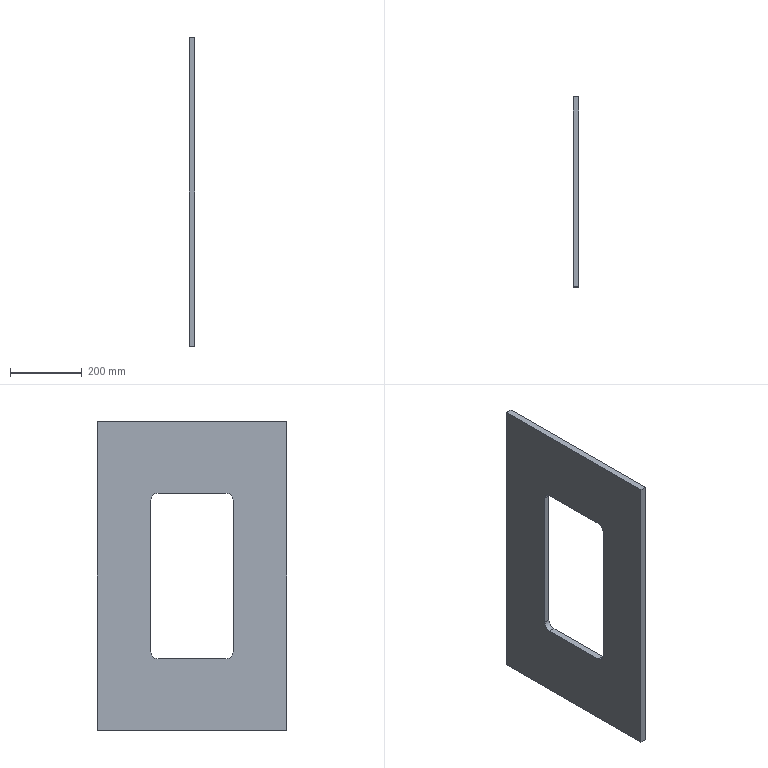Component | SolidWorks | ElectromagneticBeamRibPlate2-1 | 1 solid | 14 faces | box 16 x 530 x 864 mm | volume 5624694 mm3 | plane 10 | cylinder 4 | commonest cylinder face diameters 40 x4 | material Plain Carbon Steel
STEP:
#1=CARTESIAN_POINT('',(-224.94,116.997,228.742));
#2=VERTEX_POINT('',#1);
#3=CARTESIAN_POINT('',(-224.94,116.997,262.758));
#4=VERTEX_POINT('',#3);
#5=CARTESIAN_POINT('',(-224.94,116.997,228.742));
#6=DIRECTION('',(-0.,0.,1.));
#7=VECTOR('',#6,39.37);
#8=LINE('',#5,#7);
#9=EDGE_CURVE('',#2,#4,#8,.T.);
#10=ORIENTED_EDGE('',*,*,#9,.F.);
#11=CARTESIAN_POINT('',(-224.31,116.997,228.742));
#12=VERTEX_POINT('',#11);
#13=CARTESIAN_POINT('',(-224.31,116.997,228.742));
#14=DIRECTION('',(-1.,-0.,0.));
#15=VECTOR('',#14,39.37);
#16=LINE('',#13,#15);
#17=EDGE_CURVE('',#12,#2,#16,.T.);
#18=ORIENTED_EDGE('',*,*,#17,.F.);
#19=CARTESIAN_POINT('',(-224.31,116.997,262.758));
#20=VERTEX_POINT('',#19);
#21=CARTESIAN_POINT('',(-224.31,116.997,228.742));
#22=DIRECTION('',(-0.,0.,1.));
#23=VECTOR('',#22,39.37);
#24=LINE('',#21,#23);
#25=EDGE_CURVE('',#12,#20,#24,.T.);
#26=ORIENTED_EDGE('',*,*,#25,.T.);
#27=CARTESIAN_POINT('',(-224.31,116.997,262.758));
#28=DIRECTION('',(-1.,-0.,0.));
#29=VECTOR('',#28,39.37);
#30=LINE('',#27,#29);
#31=EDGE_CURVE('',#20,#4,#30,.T.);
#32=ORIENTED_EDGE('',*,*,#31,.T.);
#33=EDGE_LOOP('',(#10,#18,#26,#32));
#34=FACE_OUTER_BOUND('',#33,.T.);
#35=CARTESIAN_POINT('',(-224.31,116.997,228.742));
#36=DIRECTION('',(0.,-1.,0.));
#37=DIRECTION('',(-0.,0.,1.));
#38=AXIS2_PLACEMENT_3D('',#35,#36,#37);
#39=PLANE('',#38);
#40=ADVANCED_FACE('',(#34),#39,.T.);
#41=CARTESIAN_POINT('',(-224.94,137.863,228.742));
#42=VERTEX_POINT('',#41);
#43=CARTESIAN_POINT('',(-224.94,116.997,228.742));
#44=DIRECTION('',(0.,-1.,0.));
#45=VECTOR('',#44,39.37);
#46=LINE('',#43,#45);
#47=EDGE_CURVE('',#42,#2,#46,.T.);
#48=ORIENTED_EDGE('',*,*,#47,.F.);
#49=CARTESIAN_POINT('',(-224.31,137.863,228.742));
#50=VERTEX_POINT('',#49);
#51=CARTESIAN_POINT('',(-224.31,137.863,228.742));
#52=DIRECTION('',(-1.,-0.,0.));
#53=VECTOR('',#52,39.37);
#54=LINE('',#51,#53);
#55=EDGE_CURVE('',#50,#42,#54,.T.);
#56=ORIENTED_EDGE('',*,*,#55,.F.);
#57=CARTESIAN_POINT('',(-224.31,116.997,228.742));
#58=DIRECTION('',(0.,-1.,0.));
#59=VECTOR('',#58,39.37);
#60=LINE('',#57,#59);
#61=EDGE_CURVE('',#50,#12,#60,.T.);
#62=ORIENTED_EDGE('',*,*,#61,.T.);
#63=ORIENTED_EDGE('',*,*,#17,.T.);
#64=EDGE_LOOP('',(#48,#56,#62,#63));
#65=FACE_OUTER_BOUND('',#64,.T.);
#66=CARTESIAN_POINT('',(-224.31,116.997,228.742));
#67=DIRECTION('',(0.,0.,-1.));
#68=DIRECTION('',(0.,-1.,0.));
#69=AXIS2_PLACEMENT_3D('',#66,#67,#68);
#70=PLANE('',#69);
#71=ADVANCED_FACE('',(#65),#70,.T.);
#72=CARTESIAN_POINT('',(-224.94,137.863,262.758));
#73=VERTEX_POINT('',#72);
#74=CARTESIAN_POINT('',(-224.94,137.863,228.742));
#75=DIRECTION('',(0.,-0.,-1.));
#76=VECTOR('',#75,39.37);
#77=LINE('',#74,#76);
#78=EDGE_CURVE('',#73,#42,#77,.T.);
#79=ORIENTED_EDGE('',*,*,#78,.F.);
#80=CARTESIAN_POINT('',(-224.31,137.863,262.758));
#81=VERTEX_POINT('',#80);
#82=CARTESIAN_POINT('',(-224.31,137.863,262.758));
#83=DIRECTION('',(-1.,-0.,0.));
#84=VECTOR('',#83,39.37);
#85=LINE('',#82,#84);
#86=EDGE_CURVE('',#81,#73,#85,.T.);
#87=ORIENTED_EDGE('',*,*,#86,.F.);
#88=CARTESIAN_POINT('',(-224.31,137.863,228.742));
#89=DIRECTION('',(0.,-0.,-1.));
#90=VECTOR('',#89,39.37);
#91=LINE('',#88,#90);
#92=EDGE_CURVE('',#81,#50,#91,.T.);
#93=ORIENTED_EDGE('',*,*,#92,.T.);
#94=ORIENTED_EDGE('',*,*,#55,.T.);
#95=EDGE_LOOP('',(#79,#87,#93,#94));
#96=FACE_OUTER_BOUND('',#95,.T.);
#97=CARTESIAN_POINT('',(-224.31,137.863,228.742));
#98=DIRECTION('',(-0.,1.,-0.));
#99=DIRECTION('',(0.,-0.,-1.));
#100=AXIS2_PLACEMENT_3D('',#97,#98,#99);
#101=PLANE('',#100);
#102=ADVANCED_FACE('',(#96),#101,.T.);
#103=CARTESIAN_POINT('',(-224.94,116.997,262.758));
#104=DIRECTION('',(-0.,1.,0.));
#105=VECTOR('',#104,39.37);
#106=LINE('',#103,#105);
#107=EDGE_CURVE('',#4,#73,#106,.T.);
#108=ORIENTED_EDGE('',*,*,#107,.F.);
#109=ORIENTED_EDGE('',*,*,#31,.F.);
#110=CARTESIAN_POINT('',(-224.31,116.997,262.758));
#111=DIRECTION('',(-0.,1.,0.));
#112=VECTOR('',#111,39.37);
#113=LINE('',#110,#112);
#114=EDGE_CURVE('',#20,#81,#113,.T.);
#115=ORIENTED_EDGE('',*,*,#114,.T.);
#116=ORIENTED_EDGE('',*,*,#86,.T.);
#117=EDGE_LOOP('',(#108,#109,#115,#116));
#118=FACE_OUTER_BOUND('',#117,.T.);
#119=CARTESIAN_POINT('',(-224.31,116.997,262.758));
#120=DIRECTION('',(0.,0.,1.));
#121=DIRECTION('',(-0.,1.,0.));
#122=AXIS2_PLACEMENT_3D('',#119,#120,#121);
#123=PLANE('',#122);
#124=ADVANCED_FACE('',(#118),#123,.T.);
#125=CARTESIAN_POINT('',(-224.31,122.903,237.403));
#126=VERTEX_POINT('',#125);
#127=CARTESIAN_POINT('',(-224.31,122.903,254.096));
#128=VERTEX_POINT('',#127);
#129=CARTESIAN_POINT('',(-224.31,122.903,237.403));
#130=DIRECTION('',(-0.,0.,1.));
#131=VECTOR('',#130,39.37);
#132=LINE('',#129,#131);
#133=EDGE_CURVE('',#126,#128,#132,.T.);
#134=ORIENTED_EDGE('',*,*,#133,.T.);
#135=CARTESIAN_POINT('',(-224.31,123.69,254.884));
#136=VERTEX_POINT('',#135);
#137=CARTESIAN_POINT('',(-224.31,123.69,254.096));
#138=DIRECTION('',(-1.,-0.,0.));
#139=DIRECTION('',(0.,0.,1.));
#140=AXIS2_PLACEMENT_3D('',#137,#138,#139);
#141=CIRCLE('',#140,0.7874);
#142=EDGE_CURVE('',#128,#136,#141,.T.);
#143=ORIENTED_EDGE('',*,*,#142,.T.);
#144=CARTESIAN_POINT('',(-224.31,131.171,254.884));
#145=VERTEX_POINT('',#144);
#146=CARTESIAN_POINT('',(-224.31,123.69,254.884));
#147=DIRECTION('',(-0.,1.,0.));
#148=VECTOR('',#147,39.37);
#149=LINE('',#146,#148);
#150=EDGE_CURVE('',#136,#145,#149,.T.);
#151=ORIENTED_EDGE('',*,*,#150,.T.);
#152=CARTESIAN_POINT('',(-224.31,131.958,254.096));
#153=VERTEX_POINT('',#152);
#154=CARTESIAN_POINT('',(-224.31,131.171,254.096));
#155=DIRECTION('',(-1.,-0.,0.));
#156=DIRECTION('',(0.,0.,1.));
#157=AXIS2_PLACEMENT_3D('',#154,#155,#156);
#158=CIRCLE('',#157,0.7874);
#159=EDGE_CURVE('',#145,#153,#158,.T.);
#160=ORIENTED_EDGE('',*,*,#159,.T.);
#161=CARTESIAN_POINT('',(-224.31,131.958,237.403));
#162=VERTEX_POINT('',#161);
#163=CARTESIAN_POINT('',(-224.31,131.958,237.403));
#164=DIRECTION('',(0.,-0.,-1.));
#165=VECTOR('',#164,39.37);
#166=LINE('',#163,#165);
#167=EDGE_CURVE('',#153,#162,#166,.T.);
#168=ORIENTED_EDGE('',*,*,#167,.T.);
#169=CARTESIAN_POINT('',(-224.31,131.171,236.616));
#170=VERTEX_POINT('',#169);
#171=CARTESIAN_POINT('',(-224.31,131.171,237.403));
#172=DIRECTION('',(-1.,-0.,0.));
#173=DIRECTION('',(0.,0.,-1.));
#174=AXIS2_PLACEMENT_3D('',#171,#172,#173);
#175=CIRCLE('',#174,0.7874);
#176=EDGE_CURVE('',#162,#170,#175,.T.);
#177=ORIENTED_EDGE('',*,*,#176,.T.);
#178=CARTESIAN_POINT('',(-224.31,123.69,236.616));
#179=VERTEX_POINT('',#178);
#180=CARTESIAN_POINT('',(-224.31,123.69,236.616));
#181=DIRECTION('',(0.,-1.,0.));
#182=VECTOR('',#181,39.37);
#183=LINE('',#180,#182);
#184=EDGE_CURVE('',#170,#179,#183,.T.);
#185=ORIENTED_EDGE('',*,*,#184,.T.);
#186=CARTESIAN_POINT('',(-224.31,123.69,237.403));
#187=DIRECTION('',(-1.,-0.,0.));
#188=DIRECTION('',(0.,0.,1.));
#189=AXIS2_PLACEMENT_3D('',#186,#187,#188);
#190=CIRCLE('',#189,0.7874);
#191=EDGE_CURVE('',#179,#126,#190,.T.);
#192=ORIENTED_EDGE('',*,*,#191,.T.);
#193=EDGE_LOOP('',(#134,#143,#151,#160,#168,#177,#185,#192));
#194=FACE_BOUND('',#193,.T.);
#195=ORIENTED_EDGE('',*,*,#25,.F.);
#196=ORIENTED_EDGE('',*,*,#61,.F.);
#197=ORIENTED_EDGE('',*,*,#92,.F.);
#198=ORIENTED_EDGE('',*,*,#114,.F.);
#199=EDGE_LOOP('',(#195,#196,#197,#198));
#200=FACE_OUTER_BOUND('',#199,.T.);
#201=CARTESIAN_POINT('',(-224.31,116.997,228.742));
#202=DIRECTION('',(-1.,-0.,0.));
#203=DIRECTION('',(0.,0.,1.));
#204=AXIS2_PLACEMENT_3D('',#201,#202,#203);
#205=PLANE('',#204);
#206=ADVANCED_FACE('',(#194,#200),#205,.F.);
#207=CARTESIAN_POINT('',(-224.94,122.903,254.096));
#208=VERTEX_POINT('',#207);
#209=CARTESIAN_POINT('',(-224.94,123.69,254.884));
#210=VERTEX_POINT('',#209);
#211=CARTESIAN_POINT('',(-224.94,123.69,254.096));
#212=DIRECTION('',(-1.,-0.,0.));
#213=DIRECTION('',(0.,0.,1.));
#214=AXIS2_PLACEMENT_3D('',#211,#212,#213);
#215=CIRCLE('',#214,0.7874);
#216=EDGE_CURVE('',#208,#210,#215,.T.);
#217=ORIENTED_EDGE('',*,*,#216,.F.);
#218=CARTESIAN_POINT('',(-224.94,122.903,237.403));
#219=VERTEX_POINT('',#218);
#220=CARTESIAN_POINT('',(-224.94,122.903,237.403));
#221=DIRECTION('',(-0.,0.,1.));
#222=VECTOR('',#221,39.37);
#223=LINE('',#220,#222);
#224=EDGE_CURVE('',#219,#208,#223,.T.);
#225=ORIENTED_EDGE('',*,*,#224,.F.);
#226=CARTESIAN_POINT('',(-224.94,123.69,236.616));
#227=VERTEX_POINT('',#226);
#228=CARTESIAN_POINT('',(-224.94,123.69,237.403));
#229=DIRECTION('',(-1.,-0.,0.));
#230=DIRECTION('',(0.,0.,1.));
#231=AXIS2_PLACEMENT_3D('',#228,#229,#230);
#232=CIRCLE('',#231,0.7874);
#233=EDGE_CURVE('',#227,#219,#232,.T.);
#234=ORIENTED_EDGE('',*,*,#233,.F.);
#235=CARTESIAN_POINT('',(-224.94,131.171,236.616));
#236=VERTEX_POINT('',#235);
#237=CARTESIAN_POINT('',(-224.94,123.69,236.616));
#238=DIRECTION('',(0.,-1.,0.));
#239=VECTOR('',#238,39.37);
#240=LINE('',#237,#239);
#241=EDGE_CURVE('',#236,#227,#240,.T.);
#242=ORIENTED_EDGE('',*,*,#241,.F.);
#243=CARTESIAN_POINT('',(-224.94,131.958,237.403));
#244=VERTEX_POINT('',#243);
#245=CARTESIAN_POINT('',(-224.94,131.171,237.403));
#246=DIRECTION('',(-1.,-0.,0.));
#247=DIRECTION('',(0.,0.,-1.));
#248=AXIS2_PLACEMENT_3D('',#245,#246,#247);
#249=CIRCLE('',#248,0.7874);
#250=EDGE_CURVE('',#244,#236,#249,.T.);
#251=ORIENTED_EDGE('',*,*,#250,.F.);
#252=CARTESIAN_POINT('',(-224.94,131.958,254.096));
#253=VERTEX_POINT('',#252);
#254=CARTESIAN_POINT('',(-224.94,131.958,237.403));
#255=DIRECTION('',(0.,-0.,-1.));
#256=VECTOR('',#255,39.37);
#257=LINE('',#254,#256);
#258=EDGE_CURVE('',#253,#244,#257,.T.);
#259=ORIENTED_EDGE('',*,*,#258,.F.);
#260=CARTESIAN_POINT('',(-224.94,131.171,254.884));
#261=VERTEX_POINT('',#260);
#262=CARTESIAN_POINT('',(-224.94,131.171,254.096));
#263=DIRECTION('',(-1.,-0.,0.));
#264=DIRECTION('',(0.,0.,1.));
#265=AXIS2_PLACEMENT_3D('',#262,#263,#264);
#266=CIRCLE('',#265,0.7874);
#267=EDGE_CURVE('',#261,#253,#266,.T.);
#268=ORIENTED_EDGE('',*,*,#267,.F.);
#269=CARTESIAN_POINT('',(-224.94,123.69,254.884));
#270=DIRECTION('',(-0.,1.,0.));
#271=VECTOR('',#270,39.37);
#272=LINE('',#269,#271);
#273=EDGE_CURVE('',#210,#261,#272,.T.);
#274=ORIENTED_EDGE('',*,*,#273,.F.);
#275=EDGE_LOOP('',(#217,#225,#234,#242,#251,#259,#268,#274));
#276=FACE_BOUND('',#275,.T.);
#277=ORIENTED_EDGE('',*,*,#9,.T.);
#278=ORIENTED_EDGE('',*,*,#107,.T.);
#279=ORIENTED_EDGE('',*,*,#78,.T.);
#280=ORIENTED_EDGE('',*,*,#47,.T.);
#281=EDGE_LOOP('',(#277,#278,#279,#280));
#282=FACE_OUTER_BOUND('',#281,.T.);
#283=CARTESIAN_POINT('',(-224.94,116.997,228.742));
#284=DIRECTION('',(-1.,-0.,0.));
#285=DIRECTION('',(0.,0.,1.));
#286=AXIS2_PLACEMENT_3D('',#283,#284,#285);
#287=PLANE('',#286);
#288=ADVANCED_FACE('',(#276,#282),#287,.T.);
#289=ORIENTED_EDGE('',*,*,#216,.T.);
#290=CARTESIAN_POINT('',(-224.31,123.69,254.884));
#291=DIRECTION('',(-1.,-0.,0.));
#292=VECTOR('',#291,39.37);
#293=LINE('',#290,#292);
#294=EDGE_CURVE('',#136,#210,#293,.T.);
#295=ORIENTED_EDGE('',*,*,#294,.F.);
#296=ORIENTED_EDGE('',*,*,#142,.F.);
#297=CARTESIAN_POINT('',(-224.31,122.903,254.096));
#298=DIRECTION('',(-1.,-0.,0.));
#299=VECTOR('',#298,39.37);
#300=LINE('',#297,#299);
#301=EDGE_CURVE('',#128,#208,#300,.T.);
#302=ORIENTED_EDGE('',*,*,#301,.T.);
#303=EDGE_LOOP('',(#289,#295,#296,#302));
#304=FACE_OUTER_BOUND('',#303,.T.);
#305=CARTESIAN_POINT('',(-224.31,123.69,254.096));
#306=DIRECTION('',(-1.,-0.,0.));
#307=DIRECTION('',(0.,0.,1.));
#308=AXIS2_PLACEMENT_3D('',#305,#306,#307);
#309=CYLINDRICAL_SURFACE('',#308,0.7874);
#310=ADVANCED_FACE('',(#304),#309,.F.);
#311=ORIENTED_EDGE('',*,*,#224,.T.);
#312=ORIENTED_EDGE('',*,*,#301,.F.);
#313=ORIENTED_EDGE('',*,*,#133,.F.);
#314=CARTESIAN_POINT('',(-224.31,122.903,237.403));
#315=DIRECTION('',(-1.,-0.,0.));
#316=VECTOR('',#315,39.37);
#317=LINE('',#314,#316);
#318=EDGE_CURVE('',#126,#219,#317,.T.);
#319=ORIENTED_EDGE('',*,*,#318,.T.);
#320=EDGE_LOOP('',(#311,#312,#313,#319));
#321=FACE_OUTER_BOUND('',#320,.T.);
#322=CARTESIAN_POINT('',(-224.31,122.903,237.403));
#323=DIRECTION('',(0.,-1.,0.));
#324=DIRECTION('',(-0.,0.,1.));
#325=AXIS2_PLACEMENT_3D('',#322,#323,#324);
#326=PLANE('',#325);
#327=ADVANCED_FACE('',(#321),#326,.F.);
#328=ORIENTED_EDGE('',*,*,#233,.T.);
#329=ORIENTED_EDGE('',*,*,#318,.F.);
#330=ORIENTED_EDGE('',*,*,#191,.F.);
#331=CARTESIAN_POINT('',(-224.31,123.69,236.616));
#332=DIRECTION('',(-1.,-0.,0.));
#333=VECTOR('',#332,39.37);
#334=LINE('',#331,#333);
#335=EDGE_CURVE('',#179,#227,#334,.T.);
#336=ORIENTED_EDGE('',*,*,#335,.T.);
#337=EDGE_LOOP('',(#328,#329,#330,#336));
#338=FACE_OUTER_BOUND('',#337,.T.);
#339=CARTESIAN_POINT('',(-224.31,123.69,237.403));
#340=DIRECTION('',(-1.,-0.,0.));
#341=DIRECTION('',(0.,0.,1.));
#342=AXIS2_PLACEMENT_3D('',#339,#340,#341);
#343=CYLINDRICAL_SURFACE('',#342,0.7874);
#344=ADVANCED_FACE('',(#338),#343,.F.);
#345=ORIENTED_EDGE('',*,*,#241,.T.);
#346=ORIENTED_EDGE('',*,*,#335,.F.);
#347=ORIENTED_EDGE('',*,*,#184,.F.);
#348=CARTESIAN_POINT('',(-224.31,131.171,236.616));
#349=DIRECTION('',(-1.,-0.,0.));
#350=VECTOR('',#349,39.37);
#351=LINE('',#348,#350);
#352=EDGE_CURVE('',#170,#236,#351,.T.);
#353=ORIENTED_EDGE('',*,*,#352,.T.);
#354=EDGE_LOOP('',(#345,#346,#347,#353));
#355=FACE_OUTER_BOUND('',#354,.T.);
#356=CARTESIAN_POINT('',(-224.31,123.69,236.616));
#357=DIRECTION('',(0.,0.,-1.));
#358=DIRECTION('',(0.,-1.,0.));
#359=AXIS2_PLACEMENT_3D('',#356,#357,#358);
#360=PLANE('',#359);
#361=ADVANCED_FACE('',(#355),#360,.F.);
#362=ORIENTED_EDGE('',*,*,#250,.T.);
#363=ORIENTED_EDGE('',*,*,#352,.F.);
#364=ORIENTED_EDGE('',*,*,#176,.F.);
#365=CARTESIAN_POINT('',(-224.31,131.958,237.403));
#366=DIRECTION('',(-1.,-0.,0.));
#367=VECTOR('',#366,39.37);
#368=LINE('',#365,#367);
#369=EDGE_CURVE('',#162,#244,#368,.T.);
#370=ORIENTED_EDGE('',*,*,#369,.T.);
#371=EDGE_LOOP('',(#362,#363,#364,#370));
#372=FACE_OUTER_BOUND('',#371,.T.);
#373=CARTESIAN_POINT('',(-224.31,131.171,237.403));
#374=DIRECTION('',(-1.,-0.,0.));
#375=DIRECTION('',(0.,0.,1.));
#376=AXIS2_PLACEMENT_3D('',#373,#374,#375);
#377=CYLINDRICAL_SURFACE('',#376,0.7874);
#378=ADVANCED_FACE('',(#372),#377,.F.);
#379=ORIENTED_EDGE('',*,*,#258,.T.);
#380=ORIENTED_EDGE('',*,*,#369,.F.);
#381=ORIENTED_EDGE('',*,*,#167,.F.);
#382=CARTESIAN_POINT('',(-224.31,131.958,254.096));
#383=DIRECTION('',(-1.,-0.,0.));
#384=VECTOR('',#383,39.37);
#385=LINE('',#382,#384);
#386=EDGE_CURVE('',#153,#253,#385,.T.);
#387=ORIENTED_EDGE('',*,*,#386,.T.);
#388=EDGE_LOOP('',(#379,#380,#381,#387));
#389=FACE_OUTER_BOUND('',#388,.T.);
#390=CARTESIAN_POINT('',(-224.31,131.958,237.403));
#391=DIRECTION('',(-0.,1.,-0.));
#392=DIRECTION('',(0.,-0.,-1.));
#393=AXIS2_PLACEMENT_3D('',#390,#391,#392);
#394=PLANE('',#393);
#395=ADVANCED_FACE('',(#389),#394,.F.);
#396=ORIENTED_EDGE('',*,*,#267,.T.);
#397=ORIENTED_EDGE('',*,*,#386,.F.);
#398=ORIENTED_EDGE('',*,*,#159,.F.);
#399=CARTESIAN_POINT('',(-224.31,131.171,254.884));
#400=DIRECTION('',(-1.,-0.,0.));
#401=VECTOR('',#400,39.37);
#402=LINE('',#399,#401);
#403=EDGE_CURVE('',#145,#261,#402,.T.);
#404=ORIENTED_EDGE('',*,*,#403,.T.);
#405=EDGE_LOOP('',(#396,#397,#398,#404));
#406=FACE_OUTER_BOUND('',#405,.T.);
#407=CARTESIAN_POINT('',(-224.31,131.171,254.096));
#408=DIRECTION('',(-1.,-0.,0.));
#409=DIRECTION('',(0.,0.,1.));
#410=AXIS2_PLACEMENT_3D('',#407,#408,#409);
#411=CYLINDRICAL_SURFACE('',#410,0.7874);
#412=ADVANCED_FACE('',(#406),#411,.F.);
#413=ORIENTED_EDGE('',*,*,#273,.T.);
#414=ORIENTED_EDGE('',*,*,#403,.F.);
#415=ORIENTED_EDGE('',*,*,#150,.F.);
#416=ORIENTED_EDGE('',*,*,#294,.T.);
#417=EDGE_LOOP('',(#413,#414,#415,#416));
#418=FACE_OUTER_BOUND('',#417,.T.);
#419=CARTESIAN_POINT('',(-224.31,123.69,254.884));
#420=DIRECTION('',(0.,0.,1.));
#421=DIRECTION('',(-0.,1.,0.));
#422=AXIS2_PLACEMENT_3D('',#419,#420,#421);
#423=PLANE('',#422);
#424=ADVANCED_FACE('',(#418),#423,.F.);
#425=CLOSED_SHELL('',(#40,#71,#102,#124,#206,#288,#310,#327,#344,#361,#378,#395,#412,#424));
#426=MANIFOLD_SOLID_BREP('',#425);
#427=CARTESIAN_POINT('',(0.,0.,0.));
#428=DIRECTION('',(0.,0.,1.));
#429=DIRECTION('',(1.,0.,0.));
#430=AXIS2_PLACEMENT_3D('',#427,#428,#429);
#431=(LENGTH_UNIT()NAMED_UNIT(*)SI_UNIT($,.METRE.));
#432=LENGTH_MEASURE_WITH_UNIT(LENGTH_MEASURE(0.0254),#431);
#433=DIMENSIONAL_EXPONENTS(1.,0.,0.,0.,0.,0.,0.);
#434=(CONVERSION_BASED_UNIT('',#432)LENGTH_UNIT()NAMED_UNIT(#433));
#435=UNCERTAINTY_MEASURE_WITH_UNIT(LENGTH_MEASURE(0.00001),#434,'','');
#436=(NAMED_UNIT(*)PLANE_ANGLE_UNIT()SI_UNIT($,.RADIAN.));
#437=(NAMED_UNIT(*)SI_UNIT($,.STERADIAN.)SOLID_ANGLE_UNIT());
#438=(GEOMETRIC_REPRESENTATION_CONTEXT(3)GLOBAL_UNCERTAINTY_ASSIGNED_CONTEXT((#435))GLOBAL_UNIT_ASSIGNED_CONTEXT((#434,#436,#437))REPRESENTATION_CONTEXT('',''));
#439=ADVANCED_BREP_SHAPE_REPRESENTATION('',(#426,#430),#438);
#440=COLOUR_RGB('',0.7922,0.8196,0.9333);
#441=FILL_AREA_STYLE_COLOUR('',#440);
#442=FILL_AREA_STYLE('',(#441));
#443=SURFACE_STYLE_FILL_AREA(#442);
#444=SURFACE_SIDE_STYLE('',(#443));
#445=SURFACE_STYLE_USAGE(.BOTH.,#444);
#446=PRESENTATION_STYLE_ASSIGNMENT((#445));
#447=STYLED_ITEM('',(#446),#426);
#448=(LENGTH_UNIT()NAMED_UNIT(*)SI_UNIT($,.METRE.));
#449=LENGTH_MEASURE_WITH_UNIT(LENGTH_MEASURE(0.0254),#448);
#450=DIMENSIONAL_EXPONENTS(1.,0.,0.,0.,0.,0.,0.);
#451=(CONVERSION_BASED_UNIT('',#449)LENGTH_UNIT()NAMED_UNIT(#450));
#452=UNCERTAINTY_MEASURE_WITH_UNIT(LENGTH_MEASURE(0.00001),#451,'','');
#453=(NAMED_UNIT(*)PLANE_ANGLE_UNIT()SI_UNIT($,.RADIAN.));
#454=(NAMED_UNIT(*)SI_UNIT($,.STERADIAN.)SOLID_ANGLE_UNIT());
#455=(GEOMETRIC_REPRESENTATION_CONTEXT(3)GLOBAL_UNCERTAINTY_ASSIGNED_CONTEXT((#452))GLOBAL_UNIT_ASSIGNED_CONTEXT((#451,#453,#454))REPRESENTATION_CONTEXT('',''));
#456=MECHANICAL_DESIGN_GEOMETRIC_PRESENTATION_REPRESENTATION('',(#447),#455);
#457=PRESENTATION_LAYER_ASSIGNMENT('','',(#447));